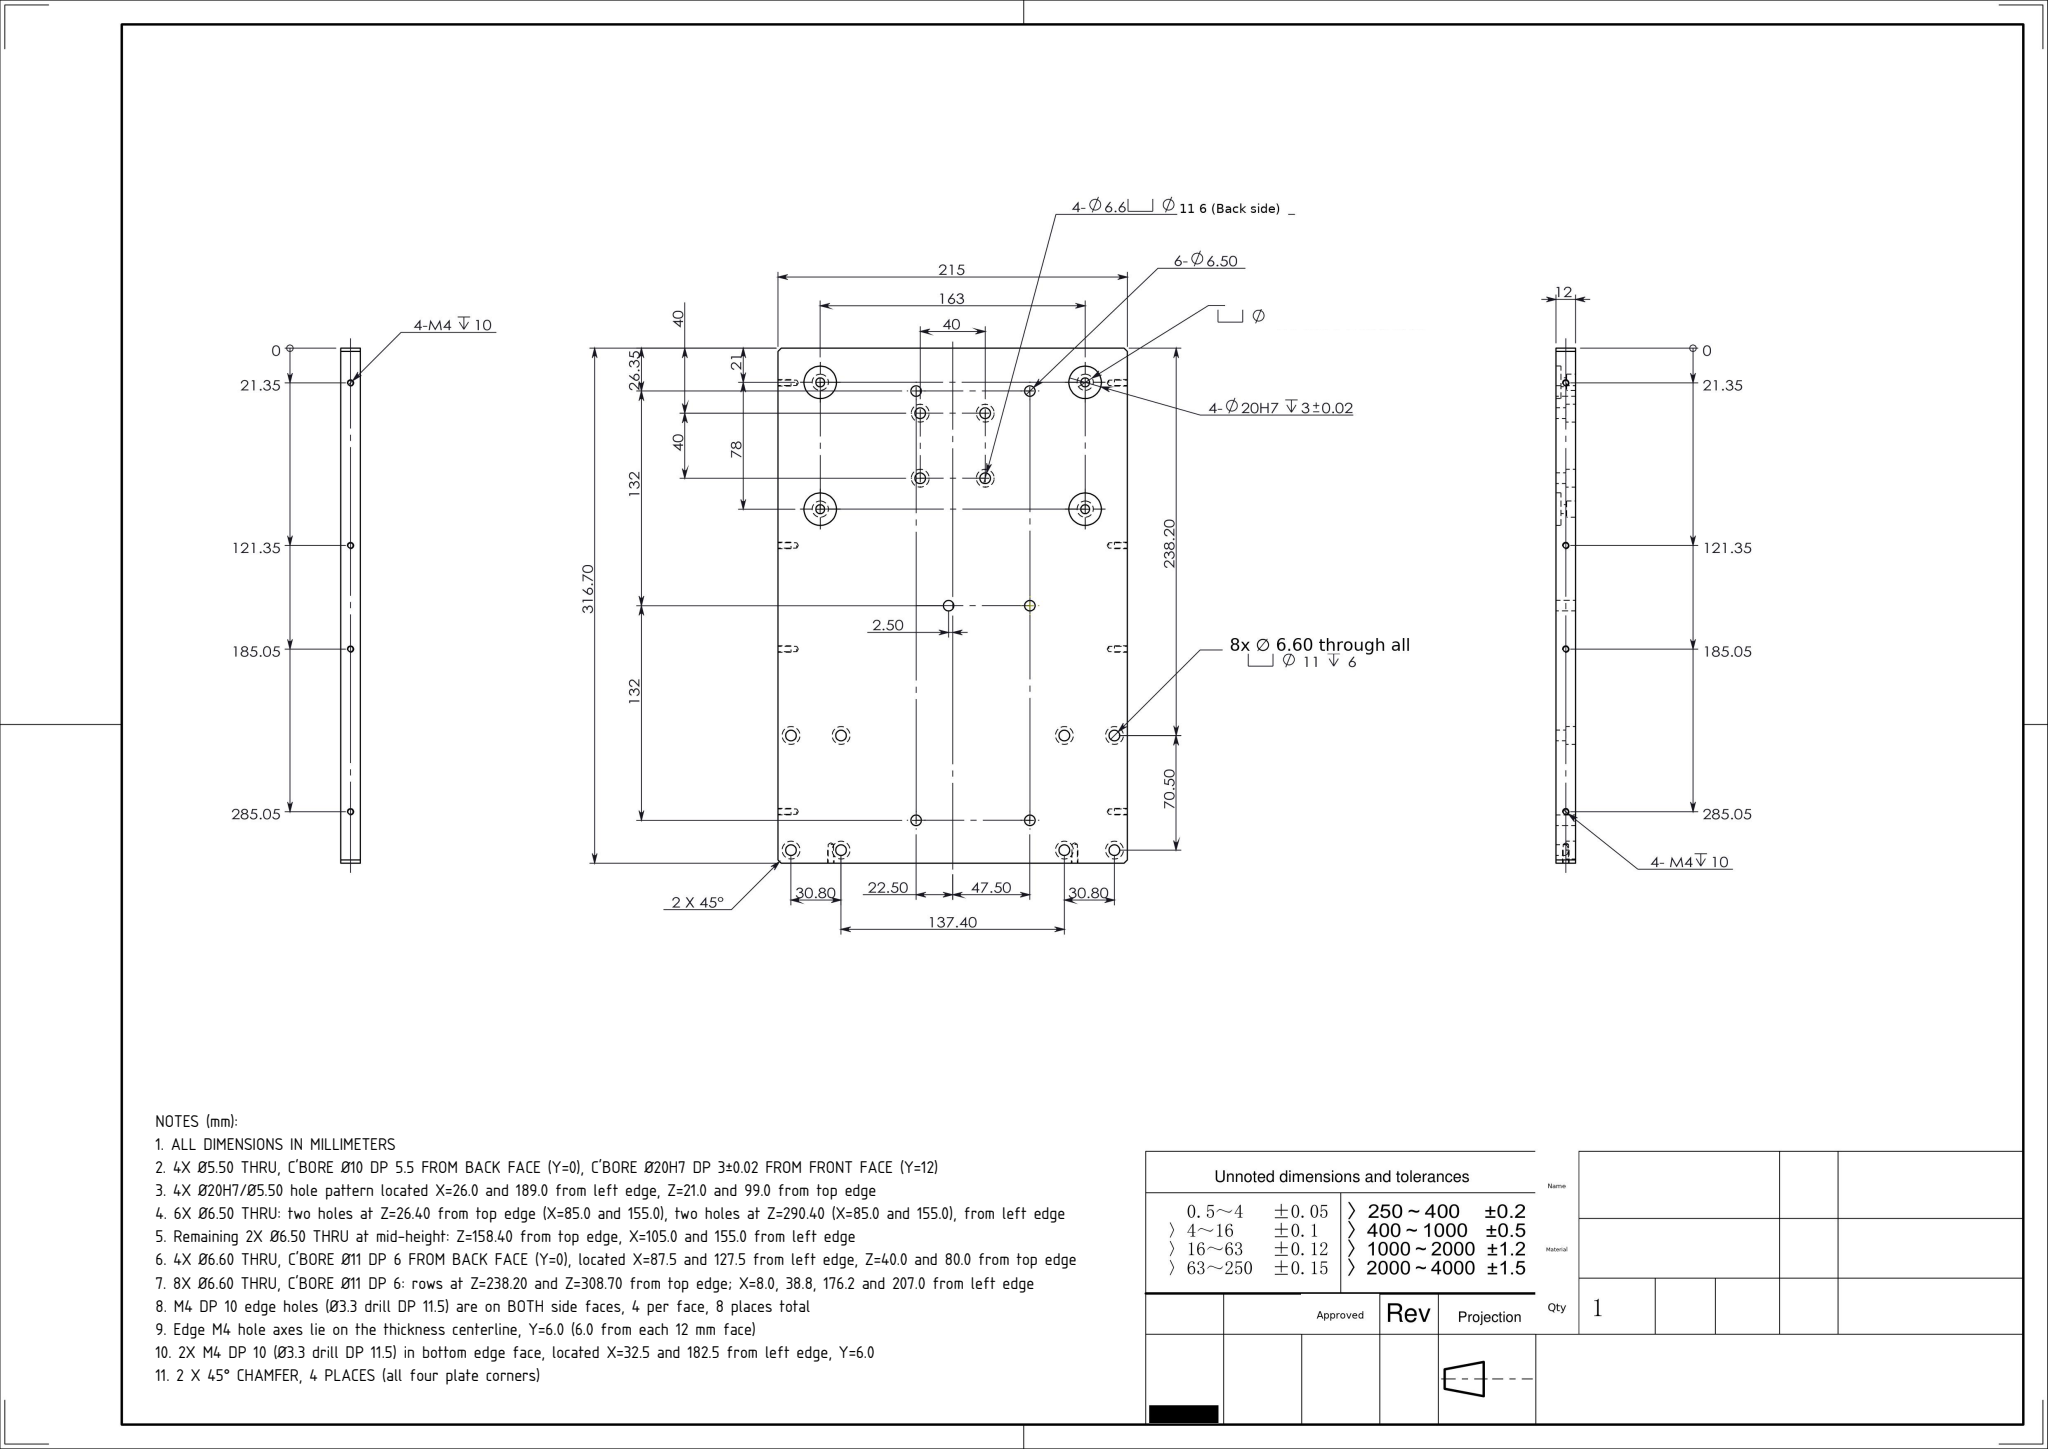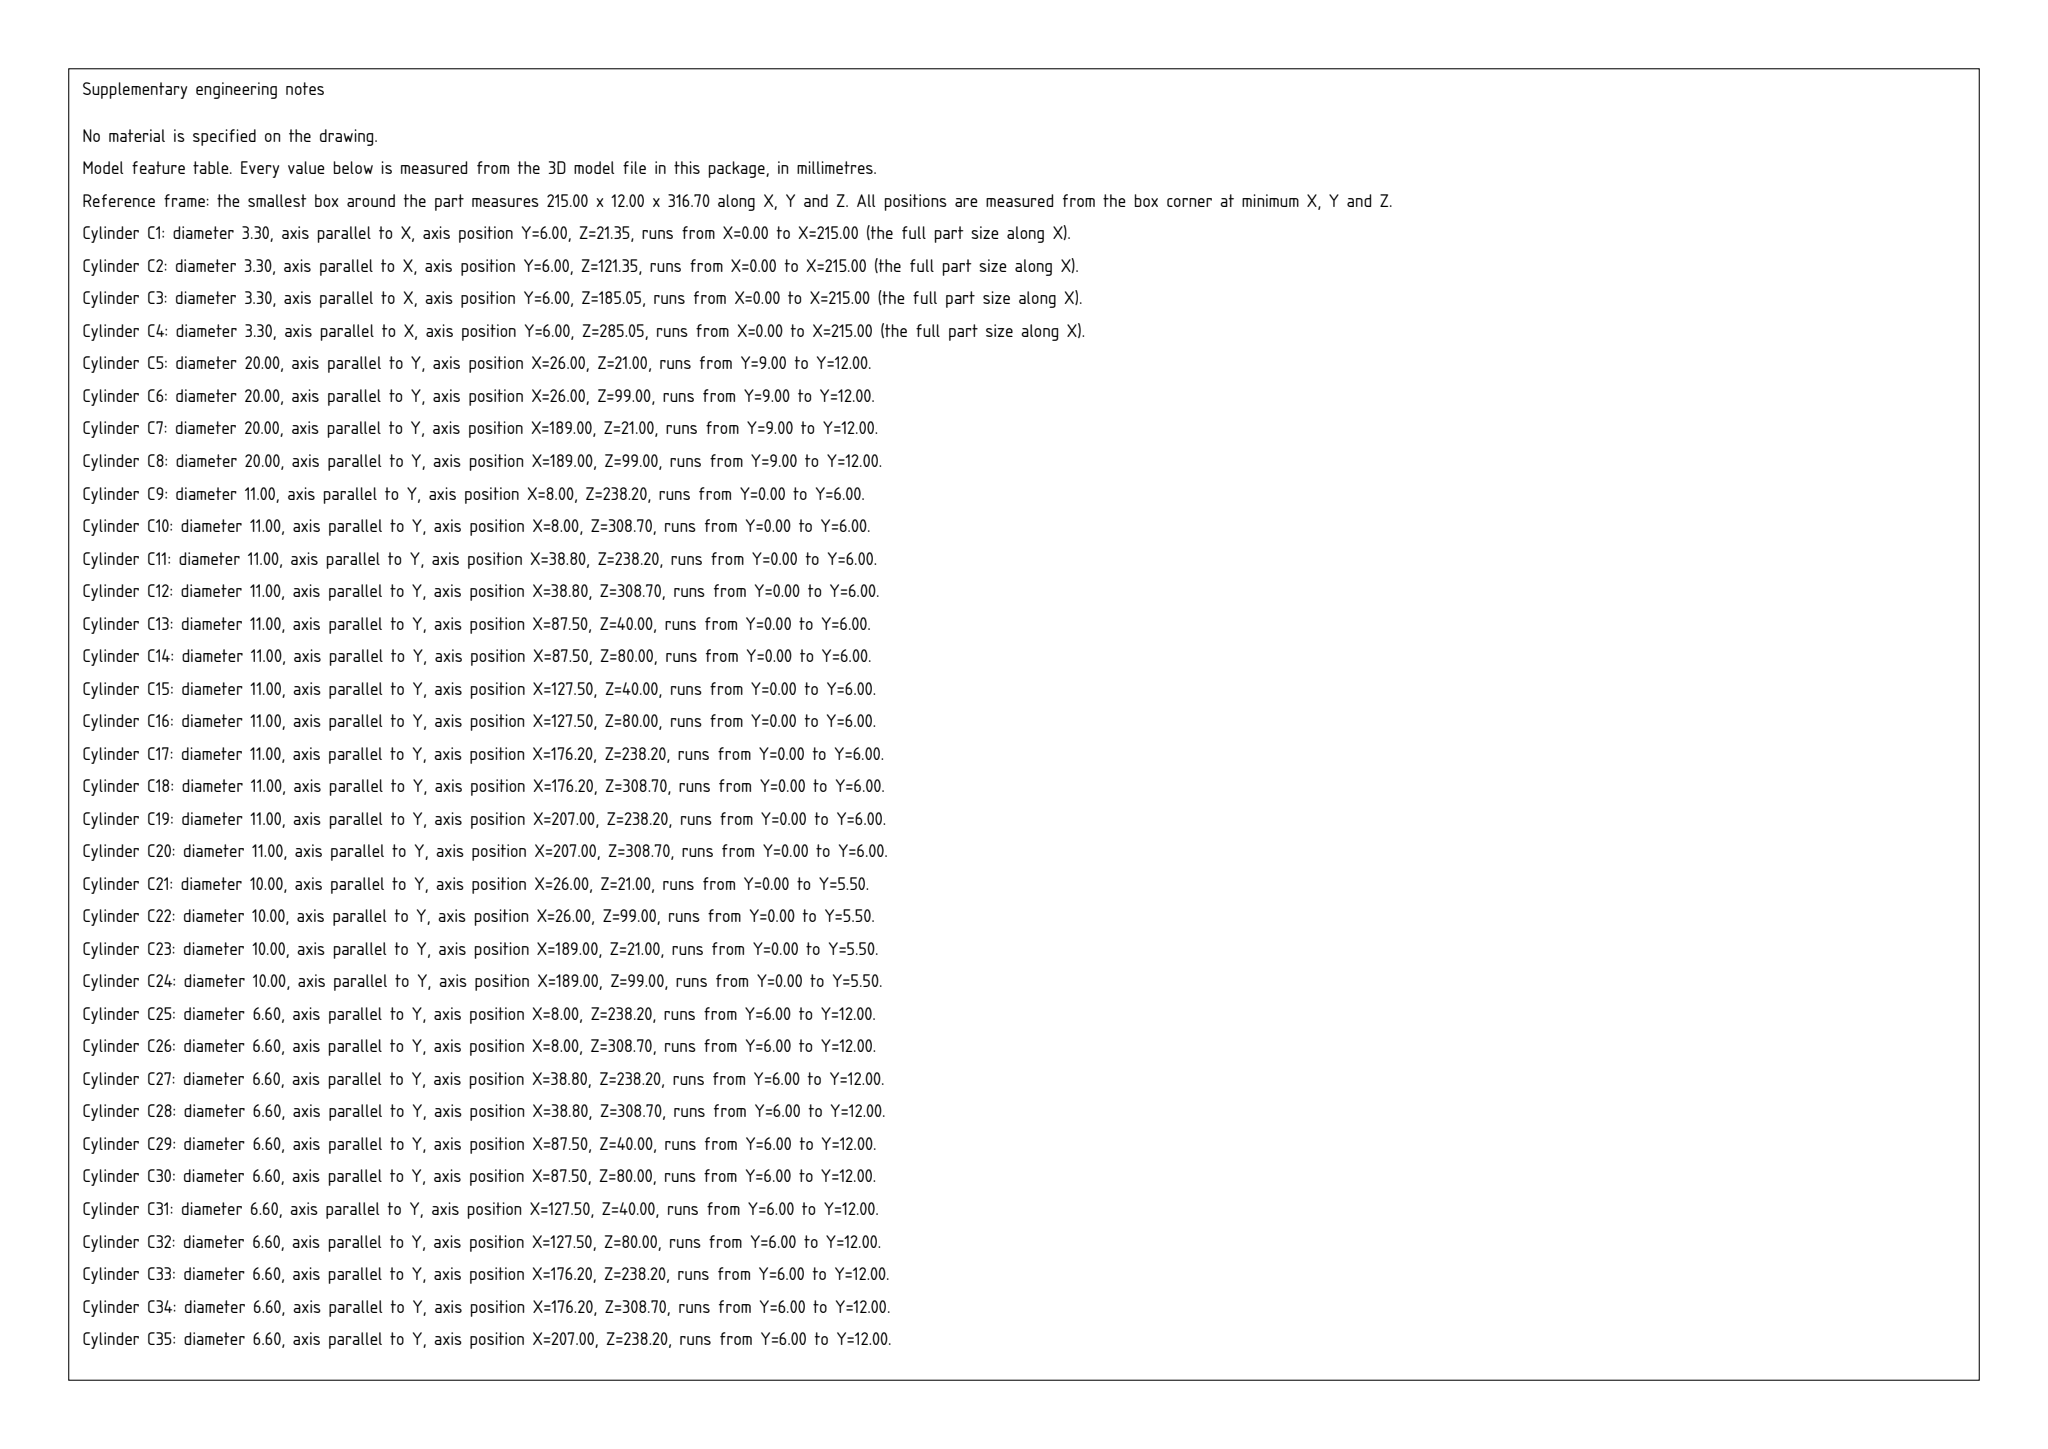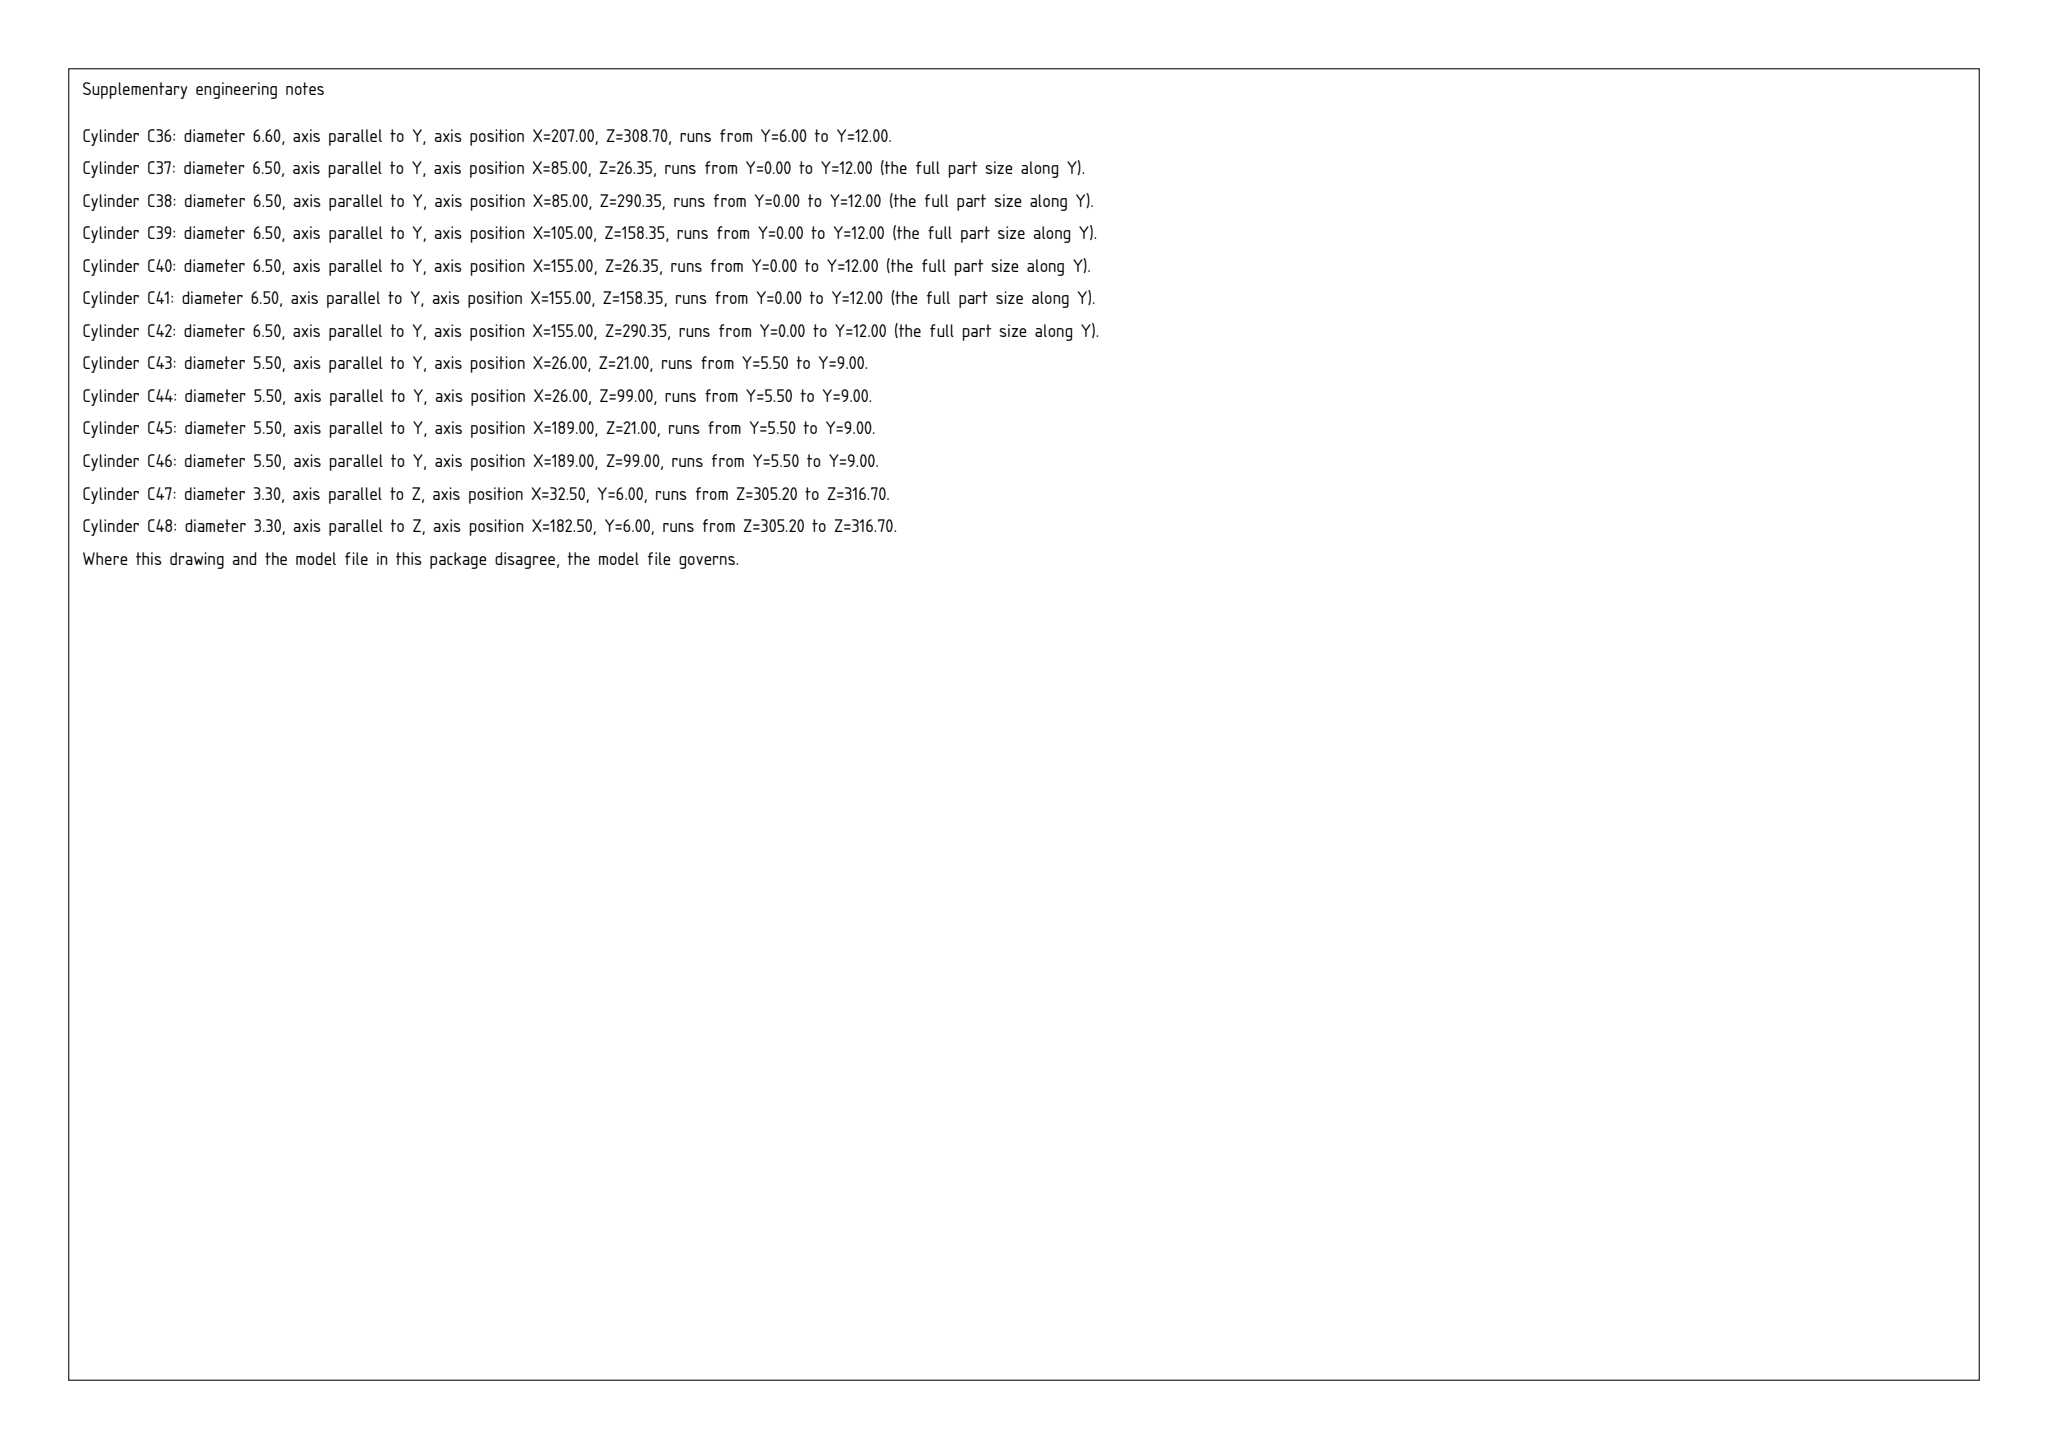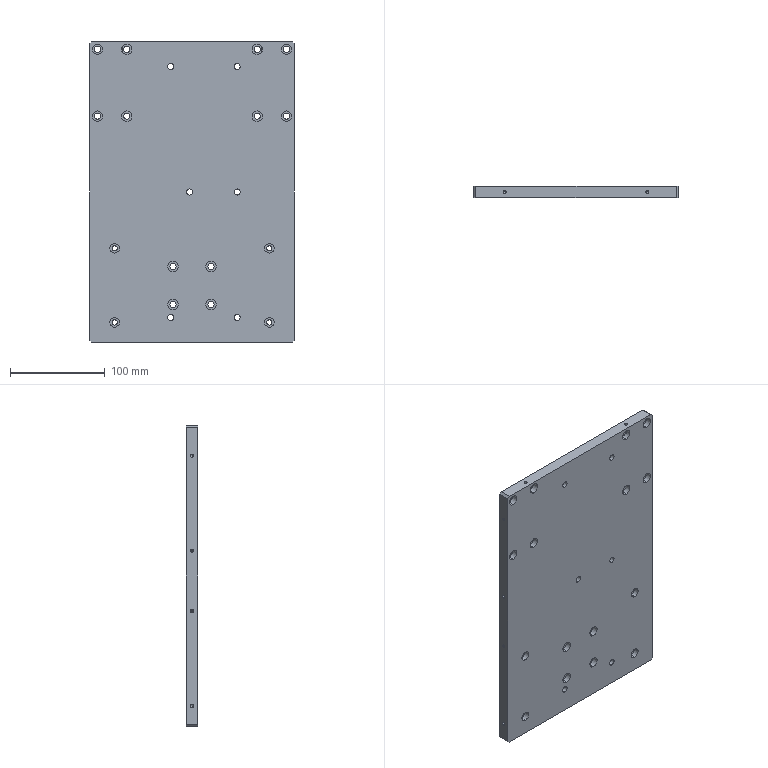Part | SolidWorks | mm | 1 solid | 154 faces | box 215 x 12 x 316.7 mm | volume 798459 mm3 | cylinder 104 | plane 30 | cone 20 | commonest cylinder face diameters 11 x24 6.6 x24 3.3 x20 6.5 x12 20 x8 10 x8 5.5 x8
Drawing notes:
ALL DIMENSIONS IN MILLIMETERS | from the solid: STEP model units mm; bbox_xyz [215.0, 12.0, 316.7]
4X Ø5.50 THRU, C'BORE Ø10 DP 5.5 FROM BACK FACE (Y=0), C'BORE Ø20H7 DP 3±0.02 FROM FRONT FACE (Y=12) | from the solid: coaxial cylinders dia 10 (y 0-5.5), dia 5.5 (y 5.5-9.0), dia 20 (y 9.0-12.0) at same XZ
4X Ø20H7/Ø5.50 hole pattern located X=26.0 and 189.0 from left edge, Z=21.0 and 99.0 from top edge | from the solid: cylinders dia 20.0, axis y, at (26,21),(26,99),(189,21),(189,99)
6X Ø6.50 THRU: two holes at Z=26.40 from top edge (X=85.0 and 155.0), two holes at Z=290.40 (X=85.0 and 155.0), from left edge | from the solid: cylinders dia 6.5, axis y, at (85,26.4),(155,26.4),(85,290.4),(155,290.4), y 0-12
Remaining 2X Ø6.50 THRU at mid-height: Z=158.40 from top edge, X=105.0 and 155.0 from left edge | from the solid: cylinders dia 6.5, axis y, at (105,158.4),(155,158.4), y 0-12
4X Ø6.60 THRU, C'BORE Ø11 DP 6 FROM BACK FACE (Y=0), located X=87.5 and 127.5 from left edge, Z=40.0 and 80.0 from top edge | from the solid: cylinders dia 11 (y 0-6) and dia 6.6 (y 6-12) at (87.5,40),(87.5,80),(127.5,40),(127.5,80)
8X Ø6.60 THRU, C'BORE Ø11 DP 6: rows at Z=238.20 and Z=308.70 from top edge; X=8.0, 38.8, 176.2 and 207.0 from left edge | from the solid: cylinders dia 11 (y 0-6) and dia 6.6 (y 6-12) at (8,238.2),(38.8,238.2),(176.2,238.2),(207,238.2),(8,308.7),(38.8,308.7),(176.2,308.7),(207,308.7)
M4 DP 10 edge holes (Ø3.3 drill DP 11.5) are on BOTH side faces, 4 per face, 8 places total | from the solid: cylinders dia 3.3, axis x, at z=21.4,121.4,185.1,285.1 for x 0-11.5 and x 203.5-215.0
Edge M4 hole axes lie on the thickness centerline, Y=6.0 (6.0 from each 12 mm face) | from the solid: cylinders dia 3.3, axis x and axis z, axis_pos y = 6.0; plate faces at y=0 and y=12
2X M4 DP 10 (Ø3.3 drill DP 11.5) in bottom edge face, located X=32.5 and 182.5 from left edge, Y=6.0 | from the solid: cylinders dia 3.3, axis z, at (32.5,6.0) and (182.5,6.0), z 305.2-316.7
2 X 45° CHAMFER, 4 PLACES (all four plate corners) | from the solid: inclined_planes: four 45° faces, size [2.0,12.0,2.0] at corners (0,0,0),(0,0,314.7),(213,0,0),(213,0,314.7)
build123d program:
from build123d import *

# Parameters (mm, degrees)
SKETCH1_W                                       = 215
SKETCH1_H                                       = 316.7
BOSS_EXTRUDE1_DEPTH                             = 12
M5_HEX_SOCKET_HEAD_CAP_SCREW_CBORE1_D           = 5.5
M5_HEX_SOCKET_HEAD_CAP_SCREW_CBORE1_CBORE_D     = 10
M5_HEX_SOCKET_HEAD_CAP_SCREW_CBORE1_CBORE_DEPTH = 5.5
SKETCH4_R                                       = 10
CUT_EXTRUDE1_DEPTH                              = 3
M6_HEX_SOCKET_HEAD_CAP_SCREW_CBORE1_D           = 6.6
M6_HEX_SOCKET_HEAD_CAP_SCREW_CBORE1_CBORE_D     = 11
M6_HEX_SOCKET_HEAD_CAP_SCREW_CBORE1_CBORE_DEPTH = 6
CHAMFER1_SIZE                                   = 2
SKETCH10_R                                      = 3.25
CUT_EXTRUDE3_DEPTH                              = 383.972
M6_HEX_SOCKET_HEAD_CAP_SCREW_CBORE3_D           = 6.6
M6_HEX_SOCKET_HEAD_CAP_SCREW_CBORE3_CBORE_D     = 11
M6_HEX_SOCKET_HEAD_CAP_SCREW_CBORE3_CBORE_DEPTH = 6
M4_TAPPED_HOLE1_D                               = 3.3
M4_TAPPED_HOLE1_DEPTH                           = 11.5
M4_TAPPED_HOLE1_TIP                             = 0.9914
M4_TAPPED_HOLE2_D                               = 3.3
M4_TAPPED_HOLE2_DEPTH                           = 11.5
M4_TAPPED_HOLE2_TIP                             = 0.9914
M4_TAPPED_HOLE3_D                               = 3.3
M4_TAPPED_HOLE3_DEPTH                           = 11.5
M4_TAPPED_HOLE3_TIP                             = 0.9914


with BuildPart() as part:
    # Sketch1 → Boss-Extrude1 (new body)
    with BuildSketch(Plane(origin=(0, 0, 0), x_dir=(1, 0, 0), z_dir=(0, 1, 0))):
        with Locations((107.5, 158.35)):
            Rectangle(SKETCH1_W, SKETCH1_H)
    extrude(amount=BOSS_EXTRUDE1_DEPTH)

    # M5 Hex Socket Head Cap Screw CBORE1 (through all)
    with Locations(Plane.XZ):
        with Locations((189, -217.7), (189, -295.7), (26, -295.7), (26, -217.7)):
            CounterBoreHole(M5_HEX_SOCKET_HEAD_CAP_SCREW_CBORE1_D / 2, M5_HEX_SOCKET_HEAD_CAP_SCREW_CBORE1_CBORE_D / 2, M5_HEX_SOCKET_HEAD_CAP_SCREW_CBORE1_CBORE_DEPTH)

    # Sketch4 → Cut-Extrude1 (cut)
    with BuildSketch(Plane(origin=(0, 12, 0), x_dir=(-1, 0, 0), z_dir=(0, 1, 0))):
        with Locations(Location((-26, -295.7, 0), (0, 0, 90))):
            Circle(SKETCH4_R)
        with Locations(Location((-26, -217.7, 0), (0, 0, 90))):
            Circle(SKETCH4_R)
        with Locations(Location((-189, -295.7, 0), (0, 0, 90))):
            Circle(SKETCH4_R)
        with Locations(Location((-189, -217.7, 0), (0, 0, 90))):
            Circle(SKETCH4_R)
    extrude(amount=-CUT_EXTRUDE1_DEPTH, mode=Mode.SUBTRACT)

    # M6 Hex Socket Head Cap Screw CBORE1 (through all)
    with Locations(Plane.XZ):
        with Locations((127.5, -276.7), (87.5, -276.7), (87.5, -236.7), (127.5, -236.7)):
            CounterBoreHole(M6_HEX_SOCKET_HEAD_CAP_SCREW_CBORE1_D / 2, M6_HEX_SOCKET_HEAD_CAP_SCREW_CBORE1_CBORE_D / 2, M6_HEX_SOCKET_HEAD_CAP_SCREW_CBORE1_CBORE_DEPTH)

    # Chamfer1
    chamfer1_edges = [part.edges().sort_by_distance(p)[0] for p in [
        (0, 6, -316.7),
        (215, 6, -316.7),
        (215, 6, 0),
        (0, 6, 0),
    ]]
    chamfer(chamfer1_edges, length=CHAMFER1_SIZE)

    # Sketch10 → Cut-Extrude3 (cut, through all)
    with BuildSketch(Plane(origin=(0, 12, 0), x_dir=(-1, 0, 0), z_dir=(0, 1, 0))):
        with Locations(Location((-85, -290.35, 0), (0, 0, 90))):
            Circle(SKETCH10_R)
        with Locations(Location((-155, -290.35, 0), (0, 0, 90))):
            Circle(SKETCH10_R)
        with Locations(Location((-85, -26.35, 0), (0, 0, 90))):
            Circle(SKETCH10_R)
        with Locations(Location((-155, -26.35, 0), (0, 0, 90))):
            Circle(SKETCH10_R)
        with Locations(Location((-105, -158.35, 0), (0, 0, 90))):
            Circle(SKETCH10_R)
        with Locations(Location((-155, -158.35, 0), (0, 0, 90))):
            Circle(SKETCH10_R)
    extrude(amount=-CUT_EXTRUDE3_DEPTH, mode=Mode.SUBTRACT)

    # M6 Hex Socket Head Cap Screw CBORE3 (through all)
    with Locations(Plane(origin=(8, 0, -8), x_dir=(0, 0, -1), z_dir=(0, -1, 0))):
        with Locations((0, 0), (70.5, 0), (0, 30.8), (70.5, 30.8), (0, 168.2), (0, 199), (70.5, 168.2), (70.5, 199)):
            CounterBoreHole(M6_HEX_SOCKET_HEAD_CAP_SCREW_CBORE3_D / 2, M6_HEX_SOCKET_HEAD_CAP_SCREW_CBORE3_CBORE_D / 2, M6_HEX_SOCKET_HEAD_CAP_SCREW_CBORE3_CBORE_DEPTH)

    # M4 Tapped Hole1
    with Locations(Plane.ZY):
        with Locations((-31.65, 6), (-131.65, 6), (-195.35, 6), (-295.35, 6)):
            Hole(M4_TAPPED_HOLE1_D / 2, depth=M4_TAPPED_HOLE1_DEPTH)
            with Locations((0, 0, -(M4_TAPPED_HOLE1_DEPTH + M4_TAPPED_HOLE1_TIP / 2))):  # 118° drill point
                Cone(0, M4_TAPPED_HOLE1_D / 2, M4_TAPPED_HOLE1_TIP, mode=Mode.SUBTRACT)

    # M4 Tapped Hole2
    with Locations(Plane.XY):
        with Locations((32.5, 6), (182.5, 6)):
            Hole(M4_TAPPED_HOLE2_D / 2, depth=M4_TAPPED_HOLE2_DEPTH)
            with Locations((0, 0, -(M4_TAPPED_HOLE2_DEPTH + M4_TAPPED_HOLE2_TIP / 2))):  # 118° drill point
                Cone(0, M4_TAPPED_HOLE2_D / 2, M4_TAPPED_HOLE2_TIP, mode=Mode.SUBTRACT)

    # M4 Tapped Hole3
    with Locations(Plane(origin=(215, 0, 0), x_dir=(0, 0, -1), z_dir=(1, 0, 0))):
        with Locations((31.65, 6), (131.65, 6), (195.35, 6), (295.35, 6)):
            Hole(M4_TAPPED_HOLE3_D / 2, depth=M4_TAPPED_HOLE3_DEPTH)
            with Locations((0, 0, -(M4_TAPPED_HOLE3_DEPTH + M4_TAPPED_HOLE3_TIP / 2))):  # 118° drill point
                Cone(0, M4_TAPPED_HOLE3_D / 2, M4_TAPPED_HOLE3_TIP, mode=Mode.SUBTRACT)


solid = part.part